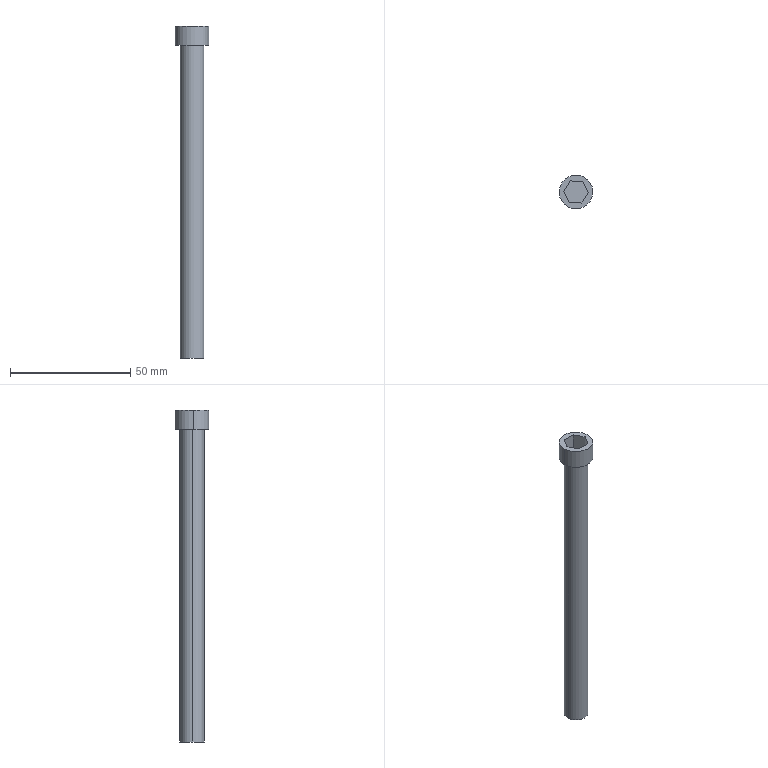Component | SolidWorks | M10Screw-1 | 1 solid | 14 faces | box 14 x 14 x 138 mm | volume 10951 mm3 | plane 10 | cylinder 4 | commonest cylinder face diameters 14 x2 10 x2
STEP:
#1=CARTESIAN_POINT('',(20.127,-9.142,63.257));
#2=VERTEX_POINT('',#1);
#3=CARTESIAN_POINT('',(19.577,-9.182,63.257));
#4=VERTEX_POINT('',#3);
#5=CARTESIAN_POINT('',(19.852,-9.162,63.257));
#6=DIRECTION('',(0.,0.,1.));
#7=DIRECTION('',(0.9975,0.07123,0.));
#8=AXIS2_PLACEMENT_3D('',#5,#6,#7);
#9=CIRCLE('',#8,0.2756);
#10=EDGE_CURVE('',#2,#4,#9,.T.);
#11=ORIENTED_EDGE('',*,*,#10,.F.);
#12=CARTESIAN_POINT('',(20.127,-9.142,62.942));
#13=VERTEX_POINT('',#12);
#14=CARTESIAN_POINT('',(20.127,-9.142,63.257));
#15=DIRECTION('',(-0.,-0.,-1.));
#16=VECTOR('',#15,39.37);
#17=LINE('',#14,#16);
#18=EDGE_CURVE('',#2,#13,#17,.T.);
#19=ORIENTED_EDGE('',*,*,#18,.T.);
#20=CARTESIAN_POINT('',(19.577,-9.182,62.942));
#21=VERTEX_POINT('',#20);
#22=CARTESIAN_POINT('',(19.852,-9.162,62.942));
#23=DIRECTION('',(0.,0.,1.));
#24=DIRECTION('',(0.9975,0.07123,0.));
#25=AXIS2_PLACEMENT_3D('',#22,#23,#24);
#26=CIRCLE('',#25,0.2756);
#27=EDGE_CURVE('',#13,#21,#26,.T.);
#28=ORIENTED_EDGE('',*,*,#27,.T.);
#29=CARTESIAN_POINT('',(19.577,-9.182,63.257));
#30=DIRECTION('',(-0.,-0.,-1.));
#31=VECTOR('',#30,39.37);
#32=LINE('',#29,#31);
#33=EDGE_CURVE('',#4,#21,#32,.T.);
#34=ORIENTED_EDGE('',*,*,#33,.F.);
#35=EDGE_LOOP('',(#11,#19,#28,#34));
#36=FACE_OUTER_BOUND('',#35,.T.);
#37=CARTESIAN_POINT('',(19.852,-9.162,63.257));
#38=DIRECTION('',(-0.,-0.,-1.));
#39=DIRECTION('',(-0.9975,-0.07123,0.));
#40=AXIS2_PLACEMENT_3D('',#37,#38,#39);
#41=CYLINDRICAL_SURFACE('',#40,0.2756);
#42=ADVANCED_FACE('',(#36),#41,.T.);
#43=CARTESIAN_POINT('',(20.048,-9.148,62.942));
#44=VERTEX_POINT('',#43);
#45=CARTESIAN_POINT('',(19.656,-9.176,62.942));
#46=VERTEX_POINT('',#45);
#47=CARTESIAN_POINT('',(19.852,-9.162,62.942));
#48=DIRECTION('',(0.,0.,1.));
#49=DIRECTION('',(0.9975,0.07123,0.));
#50=AXIS2_PLACEMENT_3D('',#47,#48,#49);
#51=CIRCLE('',#50,0.1969);
#52=EDGE_CURVE('',#44,#46,#51,.T.);
#53=ORIENTED_EDGE('',*,*,#52,.F.);
#54=CARTESIAN_POINT('',(20.048,-9.148,57.824));
#55=VERTEX_POINT('',#54);
#56=CARTESIAN_POINT('',(20.048,-9.148,62.942));
#57=DIRECTION('',(-0.,-0.,-1.));
#58=VECTOR('',#57,39.37);
#59=LINE('',#56,#58);
#60=EDGE_CURVE('',#44,#55,#59,.T.);
#61=ORIENTED_EDGE('',*,*,#60,.T.);
#62=CARTESIAN_POINT('',(19.656,-9.176,57.824));
#63=VERTEX_POINT('',#62);
#64=CARTESIAN_POINT('',(19.852,-9.162,57.824));
#65=DIRECTION('',(0.,0.,1.));
#66=DIRECTION('',(0.9975,0.07123,0.));
#67=AXIS2_PLACEMENT_3D('',#64,#65,#66);
#68=CIRCLE('',#67,0.1969);
#69=EDGE_CURVE('',#55,#63,#68,.T.);
#70=ORIENTED_EDGE('',*,*,#69,.T.);
#71=CARTESIAN_POINT('',(19.656,-9.176,62.942));
#72=DIRECTION('',(-0.,-0.,-1.));
#73=VECTOR('',#72,39.37);
#74=LINE('',#71,#73);
#75=EDGE_CURVE('',#46,#63,#74,.T.);
#76=ORIENTED_EDGE('',*,*,#75,.F.);
#77=EDGE_LOOP('',(#53,#61,#70,#76));
#78=FACE_OUTER_BOUND('',#77,.T.);
#79=CARTESIAN_POINT('',(19.852,-9.162,62.942));
#80=DIRECTION('',(-0.,-0.,-1.));
#81=DIRECTION('',(-0.9975,-0.07123,0.));
#82=AXIS2_PLACEMENT_3D('',#79,#80,#81);
#83=CYLINDRICAL_SURFACE('',#82,0.1969);
#84=ADVANCED_FACE('',(#78),#83,.T.);
#85=ORIENTED_EDGE('',*,*,#60,.F.);
#86=CARTESIAN_POINT('',(19.852,-9.162,62.942));
#87=DIRECTION('',(0.,0.,1.));
#88=DIRECTION('',(0.9975,0.07123,0.));
#89=AXIS2_PLACEMENT_3D('',#86,#87,#88);
#90=CIRCLE('',#89,0.1969);
#91=EDGE_CURVE('',#46,#44,#90,.T.);
#92=ORIENTED_EDGE('',*,*,#91,.F.);
#93=ORIENTED_EDGE('',*,*,#75,.T.);
#94=CARTESIAN_POINT('',(19.852,-9.162,57.824));
#95=DIRECTION('',(0.,0.,1.));
#96=DIRECTION('',(0.9975,0.07123,0.));
#97=AXIS2_PLACEMENT_3D('',#94,#95,#96);
#98=CIRCLE('',#97,0.1969);
#99=EDGE_CURVE('',#63,#55,#98,.T.);
#100=ORIENTED_EDGE('',*,*,#99,.T.);
#101=EDGE_LOOP('',(#85,#92,#93,#100));
#102=FACE_OUTER_BOUND('',#101,.T.);
#103=CARTESIAN_POINT('',(19.852,-9.162,62.942));
#104=DIRECTION('',(-0.,-0.,-1.));
#105=DIRECTION('',(-0.9975,-0.07123,0.));
#106=AXIS2_PLACEMENT_3D('',#103,#104,#105);
#107=CYLINDRICAL_SURFACE('',#106,0.1969);
#108=ADVANCED_FACE('',(#102),#107,.T.);
#109=ORIENTED_EDGE('',*,*,#99,.F.);
#110=ORIENTED_EDGE('',*,*,#69,.F.);
#111=EDGE_LOOP('',(#109,#110));
#112=FACE_OUTER_BOUND('',#111,.T.);
#113=CARTESIAN_POINT('',(19.852,-9.162,57.824));
#114=DIRECTION('',(0.,0.,1.));
#115=DIRECTION('',(0.9975,0.07123,-0.));
#116=AXIS2_PLACEMENT_3D('',#113,#114,#115);
#117=PLANE('',#116);
#118=ADVANCED_FACE('',(#112),#117,.F.);
#119=CARTESIAN_POINT('',(19.852,-9.162,62.942));
#120=DIRECTION('',(0.,0.,1.));
#121=DIRECTION('',(0.9975,0.07123,0.));
#122=AXIS2_PLACEMENT_3D('',#119,#120,#121);
#123=CIRCLE('',#122,0.2756);
#124=EDGE_CURVE('',#21,#13,#123,.T.);
#125=ORIENTED_EDGE('',*,*,#124,.F.);
#126=ORIENTED_EDGE('',*,*,#27,.F.);
#127=EDGE_LOOP('',(#125,#126));
#128=FACE_OUTER_BOUND('',#127,.T.);
#129=ORIENTED_EDGE('',*,*,#91,.T.);
#130=ORIENTED_EDGE('',*,*,#52,.T.);
#131=EDGE_LOOP('',(#129,#130));
#132=FACE_BOUND('',#131,.T.);
#133=CARTESIAN_POINT('',(19.852,-9.162,62.942));
#134=DIRECTION('',(0.,0.,1.));
#135=DIRECTION('',(0.9975,0.07123,-0.));
#136=AXIS2_PLACEMENT_3D('',#133,#134,#135);
#137=PLANE('',#136);
#138=ADVANCED_FACE('',(#128,#132),#137,.F.);
#139=ORIENTED_EDGE('',*,*,#18,.F.);
#140=CARTESIAN_POINT('',(19.852,-9.162,63.257));
#141=DIRECTION('',(0.,0.,1.));
#142=DIRECTION('',(0.9975,0.07123,0.));
#143=AXIS2_PLACEMENT_3D('',#140,#141,#142);
#144=CIRCLE('',#143,0.2756);
#145=EDGE_CURVE('',#4,#2,#144,.T.);
#146=ORIENTED_EDGE('',*,*,#145,.F.);
#147=ORIENTED_EDGE('',*,*,#33,.T.);
#148=ORIENTED_EDGE('',*,*,#124,.T.);
#149=EDGE_LOOP('',(#139,#146,#147,#148));
#150=FACE_OUTER_BOUND('',#149,.T.);
#151=CARTESIAN_POINT('',(19.852,-9.162,63.257));
#152=DIRECTION('',(-0.,-0.,-1.));
#153=DIRECTION('',(-0.9975,-0.07123,0.));
#154=AXIS2_PLACEMENT_3D('',#151,#152,#153);
#155=CYLINDRICAL_SURFACE('',#154,0.2756);
#156=ADVANCED_FACE('',(#150),#155,.T.);
#157=CARTESIAN_POINT('',(19.961,-8.989,63.257));
#158=VERTEX_POINT('',#157);
#159=CARTESIAN_POINT('',(19.756,-8.981,63.257));
#160=VERTEX_POINT('',#159);
#161=CARTESIAN_POINT('',(19.961,-8.989,63.257));
#162=DIRECTION('',(-0.9993,0.03756,0.));
#163=VECTOR('',#162,39.37);
#164=LINE('',#161,#163);
#165=EDGE_CURVE('',#158,#160,#164,.T.);
#166=ORIENTED_EDGE('',*,*,#165,.F.);
#167=CARTESIAN_POINT('',(20.056,-9.17,63.257));
#168=VERTEX_POINT('',#167);
#169=CARTESIAN_POINT('',(20.056,-9.17,63.257));
#170=DIRECTION('',(-0.4671,0.8842,-0.));
#171=VECTOR('',#170,39.37);
#172=LINE('',#169,#171);
#173=EDGE_CURVE('',#168,#158,#172,.T.);
#174=ORIENTED_EDGE('',*,*,#173,.F.);
#175=CARTESIAN_POINT('',(19.948,-9.343,63.257));
#176=VERTEX_POINT('',#175);
#177=CARTESIAN_POINT('',(19.948,-9.343,63.257));
#178=DIRECTION('',(0.5322,0.8466,-0.));
#179=VECTOR('',#178,39.37);
#180=LINE('',#177,#179);
#181=EDGE_CURVE('',#176,#168,#180,.T.);
#182=ORIENTED_EDGE('',*,*,#181,.F.);
#183=CARTESIAN_POINT('',(19.743,-9.335,63.257));
#184=VERTEX_POINT('',#183);
#185=CARTESIAN_POINT('',(19.743,-9.335,63.257));
#186=DIRECTION('',(0.9993,-0.03756,-0.));
#187=VECTOR('',#186,39.37);
#188=LINE('',#185,#187);
#189=EDGE_CURVE('',#184,#176,#188,.T.);
#190=ORIENTED_EDGE('',*,*,#189,.F.);
#191=CARTESIAN_POINT('',(19.648,-9.154,63.257));
#192=VERTEX_POINT('',#191);
#193=CARTESIAN_POINT('',(19.648,-9.154,63.257));
#194=DIRECTION('',(0.4671,-0.8842,0.));
#195=VECTOR('',#194,39.37);
#196=LINE('',#193,#195);
#197=EDGE_CURVE('',#192,#184,#196,.T.);
#198=ORIENTED_EDGE('',*,*,#197,.F.);
#199=CARTESIAN_POINT('',(19.756,-8.981,63.257));
#200=DIRECTION('',(-0.5322,-0.8466,0.));
#201=VECTOR('',#200,39.37);
#202=LINE('',#199,#201);
#203=EDGE_CURVE('',#160,#192,#202,.T.);
#204=ORIENTED_EDGE('',*,*,#203,.F.);
#205=EDGE_LOOP('',(#166,#174,#182,#190,#198,#204));
#206=FACE_BOUND('',#205,.T.);
#207=ORIENTED_EDGE('',*,*,#145,.T.);
#208=ORIENTED_EDGE('',*,*,#10,.T.);
#209=EDGE_LOOP('',(#207,#208));
#210=FACE_OUTER_BOUND('',#209,.T.);
#211=CARTESIAN_POINT('',(19.852,-9.162,63.257));
#212=DIRECTION('',(0.,0.,1.));
#213=DIRECTION('',(0.9975,0.07123,-0.));
#214=AXIS2_PLACEMENT_3D('',#211,#212,#213);
#215=PLANE('',#214);
#216=ADVANCED_FACE('',(#206,#210),#215,.T.);
#217=ORIENTED_EDGE('',*,*,#165,.T.);
#218=CARTESIAN_POINT('',(19.756,-8.981,62.981));
#219=VERTEX_POINT('',#218);
#220=CARTESIAN_POINT('',(19.756,-8.981,62.981));
#221=DIRECTION('',(0.,0.,1.));
#222=VECTOR('',#221,39.37);
#223=LINE('',#220,#222);
#224=EDGE_CURVE('',#219,#160,#223,.T.);
#225=ORIENTED_EDGE('',*,*,#224,.F.);
#226=CARTESIAN_POINT('',(19.961,-8.989,62.981));
#227=VERTEX_POINT('',#226);
#228=CARTESIAN_POINT('',(19.961,-8.989,62.981));
#229=DIRECTION('',(-0.9993,0.03756,0.));
#230=VECTOR('',#229,39.37);
#231=LINE('',#228,#230);
#232=EDGE_CURVE('',#227,#219,#231,.T.);
#233=ORIENTED_EDGE('',*,*,#232,.F.);
#234=CARTESIAN_POINT('',(19.961,-8.989,62.981));
#235=DIRECTION('',(0.,0.,1.));
#236=VECTOR('',#235,39.37);
#237=LINE('',#234,#236);
#238=EDGE_CURVE('',#227,#158,#237,.T.);
#239=ORIENTED_EDGE('',*,*,#238,.T.);
#240=EDGE_LOOP('',(#217,#225,#233,#239));
#241=FACE_OUTER_BOUND('',#240,.T.);
#242=CARTESIAN_POINT('',(19.961,-8.989,62.981));
#243=DIRECTION('',(0.03756,0.9993,-0.));
#244=DIRECTION('',(-0.9993,0.03756,0.));
#245=AXIS2_PLACEMENT_3D('',#242,#243,#244);
#246=PLANE('',#245);
#247=ADVANCED_FACE('',(#241),#246,.F.);
#248=ORIENTED_EDGE('',*,*,#173,.T.);
#249=ORIENTED_EDGE('',*,*,#238,.F.);
#250=CARTESIAN_POINT('',(20.056,-9.17,62.981));
#251=VERTEX_POINT('',#250);
#252=CARTESIAN_POINT('',(20.056,-9.17,62.981));
#253=DIRECTION('',(-0.4671,0.8842,-0.));
#254=VECTOR('',#253,39.37);
#255=LINE('',#252,#254);
#256=EDGE_CURVE('',#251,#227,#255,.T.);
#257=ORIENTED_EDGE('',*,*,#256,.F.);
#258=CARTESIAN_POINT('',(20.056,-9.17,62.981));
#259=DIRECTION('',(0.,0.,1.));
#260=VECTOR('',#259,39.37);
#261=LINE('',#258,#260);
#262=EDGE_CURVE('',#251,#168,#261,.T.);
#263=ORIENTED_EDGE('',*,*,#262,.T.);
#264=EDGE_LOOP('',(#248,#249,#257,#263));
#265=FACE_OUTER_BOUND('',#264,.T.);
#266=CARTESIAN_POINT('',(20.056,-9.17,62.981));
#267=DIRECTION('',(0.8842,0.4671,-0.));
#268=DIRECTION('',(-0.4671,0.8842,-0.));
#269=AXIS2_PLACEMENT_3D('',#266,#267,#268);
#270=PLANE('',#269);
#271=ADVANCED_FACE('',(#265),#270,.F.);
#272=ORIENTED_EDGE('',*,*,#181,.T.);
#273=ORIENTED_EDGE('',*,*,#262,.F.);
#274=CARTESIAN_POINT('',(19.948,-9.343,62.981));
#275=VERTEX_POINT('',#274);
#276=CARTESIAN_POINT('',(19.948,-9.343,62.981));
#277=DIRECTION('',(0.5322,0.8466,-0.));
#278=VECTOR('',#277,39.37);
#279=LINE('',#276,#278);
#280=EDGE_CURVE('',#275,#251,#279,.T.);
#281=ORIENTED_EDGE('',*,*,#280,.F.);
#282=CARTESIAN_POINT('',(19.948,-9.343,62.981));
#283=DIRECTION('',(0.,0.,1.));
#284=VECTOR('',#283,39.37);
#285=LINE('',#282,#284);
#286=EDGE_CURVE('',#275,#176,#285,.T.);
#287=ORIENTED_EDGE('',*,*,#286,.T.);
#288=EDGE_LOOP('',(#272,#273,#281,#287));
#289=FACE_OUTER_BOUND('',#288,.T.);
#290=CARTESIAN_POINT('',(19.948,-9.343,62.981));
#291=DIRECTION('',(0.8466,-0.5322,-0.));
#292=DIRECTION('',(0.5322,0.8466,-0.));
#293=AXIS2_PLACEMENT_3D('',#290,#291,#292);
#294=PLANE('',#293);
#295=ADVANCED_FACE('',(#289),#294,.F.);
#296=ORIENTED_EDGE('',*,*,#189,.T.);
#297=ORIENTED_EDGE('',*,*,#286,.F.);
#298=CARTESIAN_POINT('',(19.743,-9.335,62.981));
#299=VERTEX_POINT('',#298);
#300=CARTESIAN_POINT('',(19.743,-9.335,62.981));
#301=DIRECTION('',(0.9993,-0.03756,-0.));
#302=VECTOR('',#301,39.37);
#303=LINE('',#300,#302);
#304=EDGE_CURVE('',#299,#275,#303,.T.);
#305=ORIENTED_EDGE('',*,*,#304,.F.);
#306=CARTESIAN_POINT('',(19.743,-9.335,62.981));
#307=DIRECTION('',(0.,0.,1.));
#308=VECTOR('',#307,39.37);
#309=LINE('',#306,#308);
#310=EDGE_CURVE('',#299,#184,#309,.T.);
#311=ORIENTED_EDGE('',*,*,#310,.T.);
#312=EDGE_LOOP('',(#296,#297,#305,#311));
#313=FACE_OUTER_BOUND('',#312,.T.);
#314=CARTESIAN_POINT('',(19.743,-9.335,62.981));
#315=DIRECTION('',(-0.03756,-0.9993,0.));
#316=DIRECTION('',(0.9993,-0.03756,-0.));
#317=AXIS2_PLACEMENT_3D('',#314,#315,#316);
#318=PLANE('',#317);
#319=ADVANCED_FACE('',(#313),#318,.F.);
#320=ORIENTED_EDGE('',*,*,#197,.T.);
#321=ORIENTED_EDGE('',*,*,#310,.F.);
#322=CARTESIAN_POINT('',(19.648,-9.154,62.981));
#323=VERTEX_POINT('',#322);
#324=CARTESIAN_POINT('',(19.648,-9.154,62.981));
#325=DIRECTION('',(0.4671,-0.8842,0.));
#326=VECTOR('',#325,39.37);
#327=LINE('',#324,#326);
#328=EDGE_CURVE('',#323,#299,#327,.T.);
#329=ORIENTED_EDGE('',*,*,#328,.F.);
#330=CARTESIAN_POINT('',(19.648,-9.154,62.981));
#331=DIRECTION('',(0.,0.,1.));
#332=VECTOR('',#331,39.37);
#333=LINE('',#330,#332);
#334=EDGE_CURVE('',#323,#192,#333,.T.);
#335=ORIENTED_EDGE('',*,*,#334,.T.);
#336=EDGE_LOOP('',(#320,#321,#329,#335));
#337=FACE_OUTER_BOUND('',#336,.T.);
#338=CARTESIAN_POINT('',(19.648,-9.154,62.981));
#339=DIRECTION('',(-0.8842,-0.4671,0.));
#340=DIRECTION('',(0.4671,-0.8842,0.));
#341=AXIS2_PLACEMENT_3D('',#338,#339,#340);
#342=PLANE('',#341);
#343=ADVANCED_FACE('',(#337),#342,.F.);
#344=ORIENTED_EDGE('',*,*,#203,.T.);
#345=ORIENTED_EDGE('',*,*,#334,.F.);
#346=CARTESIAN_POINT('',(19.756,-8.981,62.981));
#347=DIRECTION('',(-0.5322,-0.8466,0.));
#348=VECTOR('',#347,39.37);
#349=LINE('',#346,#348);
#350=EDGE_CURVE('',#219,#323,#349,.T.);
#351=ORIENTED_EDGE('',*,*,#350,.F.);
#352=ORIENTED_EDGE('',*,*,#224,.T.);
#353=EDGE_LOOP('',(#344,#345,#351,#352));
#354=FACE_OUTER_BOUND('',#353,.T.);
#355=CARTESIAN_POINT('',(19.756,-8.981,62.981));
#356=DIRECTION('',(-0.8466,0.5322,0.));
#357=DIRECTION('',(-0.5322,-0.8466,0.));
#358=AXIS2_PLACEMENT_3D('',#355,#356,#357);
#359=PLANE('',#358);
#360=ADVANCED_FACE('',(#354),#359,.F.);
#361=ORIENTED_EDGE('',*,*,#232,.T.);
#362=ORIENTED_EDGE('',*,*,#350,.T.);
#363=ORIENTED_EDGE('',*,*,#328,.T.);
#364=ORIENTED_EDGE('',*,*,#304,.T.);
#365=ORIENTED_EDGE('',*,*,#280,.T.);
#366=ORIENTED_EDGE('',*,*,#256,.T.);
#367=EDGE_LOOP('',(#361,#362,#363,#364,#365,#366));
#368=FACE_OUTER_BOUND('',#367,.T.);
#369=CARTESIAN_POINT('',(19.852,-9.162,62.981));
#370=DIRECTION('',(0.,0.,1.));
#371=DIRECTION('',(0.9975,0.07123,-0.));
#372=AXIS2_PLACEMENT_3D('',#369,#370,#371);
#373=PLANE('',#372);
#374=ADVANCED_FACE('',(#368),#373,.T.);
#375=CLOSED_SHELL('',(#42,#84,#108,#118,#138,#156,#216,#247,#271,#295,#319,#343,#360,#374));
#376=MANIFOLD_SOLID_BREP('',#375);
#377=CARTESIAN_POINT('',(0.,0.,0.));
#378=DIRECTION('',(0.,0.,1.));
#379=DIRECTION('',(1.,0.,0.));
#380=AXIS2_PLACEMENT_3D('',#377,#378,#379);
#381=(LENGTH_UNIT()NAMED_UNIT(*)SI_UNIT($,.METRE.));
#382=LENGTH_MEASURE_WITH_UNIT(LENGTH_MEASURE(0.0254),#381);
#383=DIMENSIONAL_EXPONENTS(1.,0.,0.,0.,0.,0.,0.);
#384=(CONVERSION_BASED_UNIT('',#382)LENGTH_UNIT()NAMED_UNIT(#383));
#385=UNCERTAINTY_MEASURE_WITH_UNIT(LENGTH_MEASURE(0.00001),#384,'','');
#386=(NAMED_UNIT(*)PLANE_ANGLE_UNIT()SI_UNIT($,.RADIAN.));
#387=(NAMED_UNIT(*)SI_UNIT($,.STERADIAN.)SOLID_ANGLE_UNIT());
#388=(GEOMETRIC_REPRESENTATION_CONTEXT(3)GLOBAL_UNCERTAINTY_ASSIGNED_CONTEXT((#385))GLOBAL_UNIT_ASSIGNED_CONTEXT((#384,#386,#387))REPRESENTATION_CONTEXT('',''));
#389=ADVANCED_BREP_SHAPE_REPRESENTATION('',(#376,#380),#388);
#390=COLOUR_RGB('',0.7922,0.8196,0.9333);
#391=FILL_AREA_STYLE_COLOUR('',#390);
#392=FILL_AREA_STYLE('',(#391));
#393=SURFACE_STYLE_FILL_AREA(#392);
#394=SURFACE_SIDE_STYLE('',(#393));
#395=SURFACE_STYLE_USAGE(.BOTH.,#394);
#396=PRESENTATION_STYLE_ASSIGNMENT((#395));
#397=STYLED_ITEM('',(#396),#376);
#398=(LENGTH_UNIT()NAMED_UNIT(*)SI_UNIT($,.METRE.));
#399=LENGTH_MEASURE_WITH_UNIT(LENGTH_MEASURE(0.0254),#398);
#400=DIMENSIONAL_EXPONENTS(1.,0.,0.,0.,0.,0.,0.);
#401=(CONVERSION_BASED_UNIT('',#399)LENGTH_UNIT()NAMED_UNIT(#400));
#402=UNCERTAINTY_MEASURE_WITH_UNIT(LENGTH_MEASURE(0.00001),#401,'','');
#403=(NAMED_UNIT(*)PLANE_ANGLE_UNIT()SI_UNIT($,.RADIAN.));
#404=(NAMED_UNIT(*)SI_UNIT($,.STERADIAN.)SOLID_ANGLE_UNIT());
#405=(GEOMETRIC_REPRESENTATION_CONTEXT(3)GLOBAL_UNCERTAINTY_ASSIGNED_CONTEXT((#402))GLOBAL_UNIT_ASSIGNED_CONTEXT((#401,#403,#404))REPRESENTATION_CONTEXT('',''));
#406=MECHANICAL_DESIGN_GEOMETRIC_PRESENTATION_REPRESENTATION('',(#397),#405);
#407=PRESENTATION_LAYER_ASSIGNMENT('','',(#397));